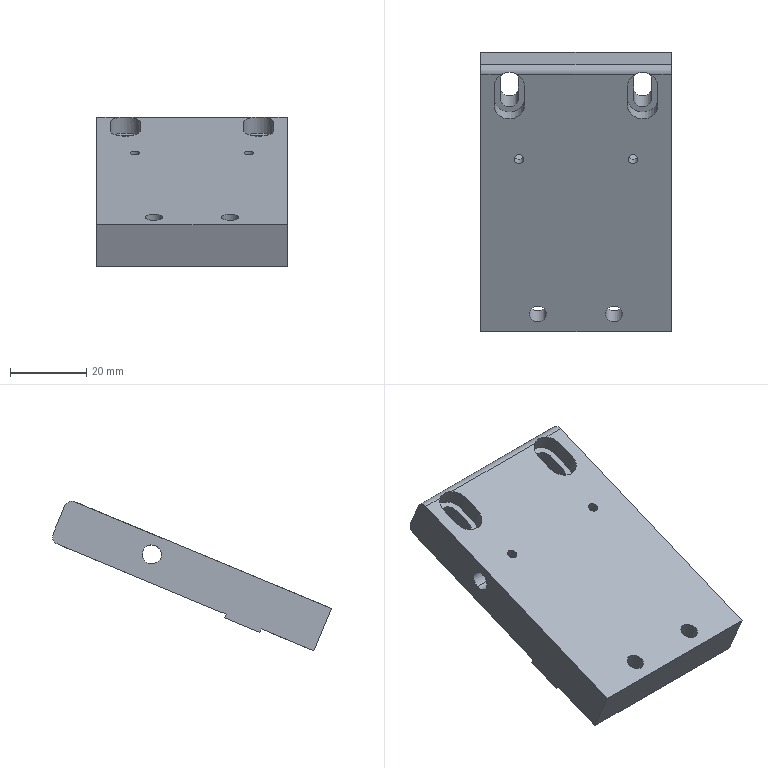Component | SolidWorks | 04-005A1MotorConnectionPlate-2 | 1 solid | 46 faces | volume 42227 mm3 | cylinder 24 | plane 22 | commonest cylinder face diameters 8 x8 2.5 x4 4.5 x4 4.8 x4 5 x2 4 x2 | material A3